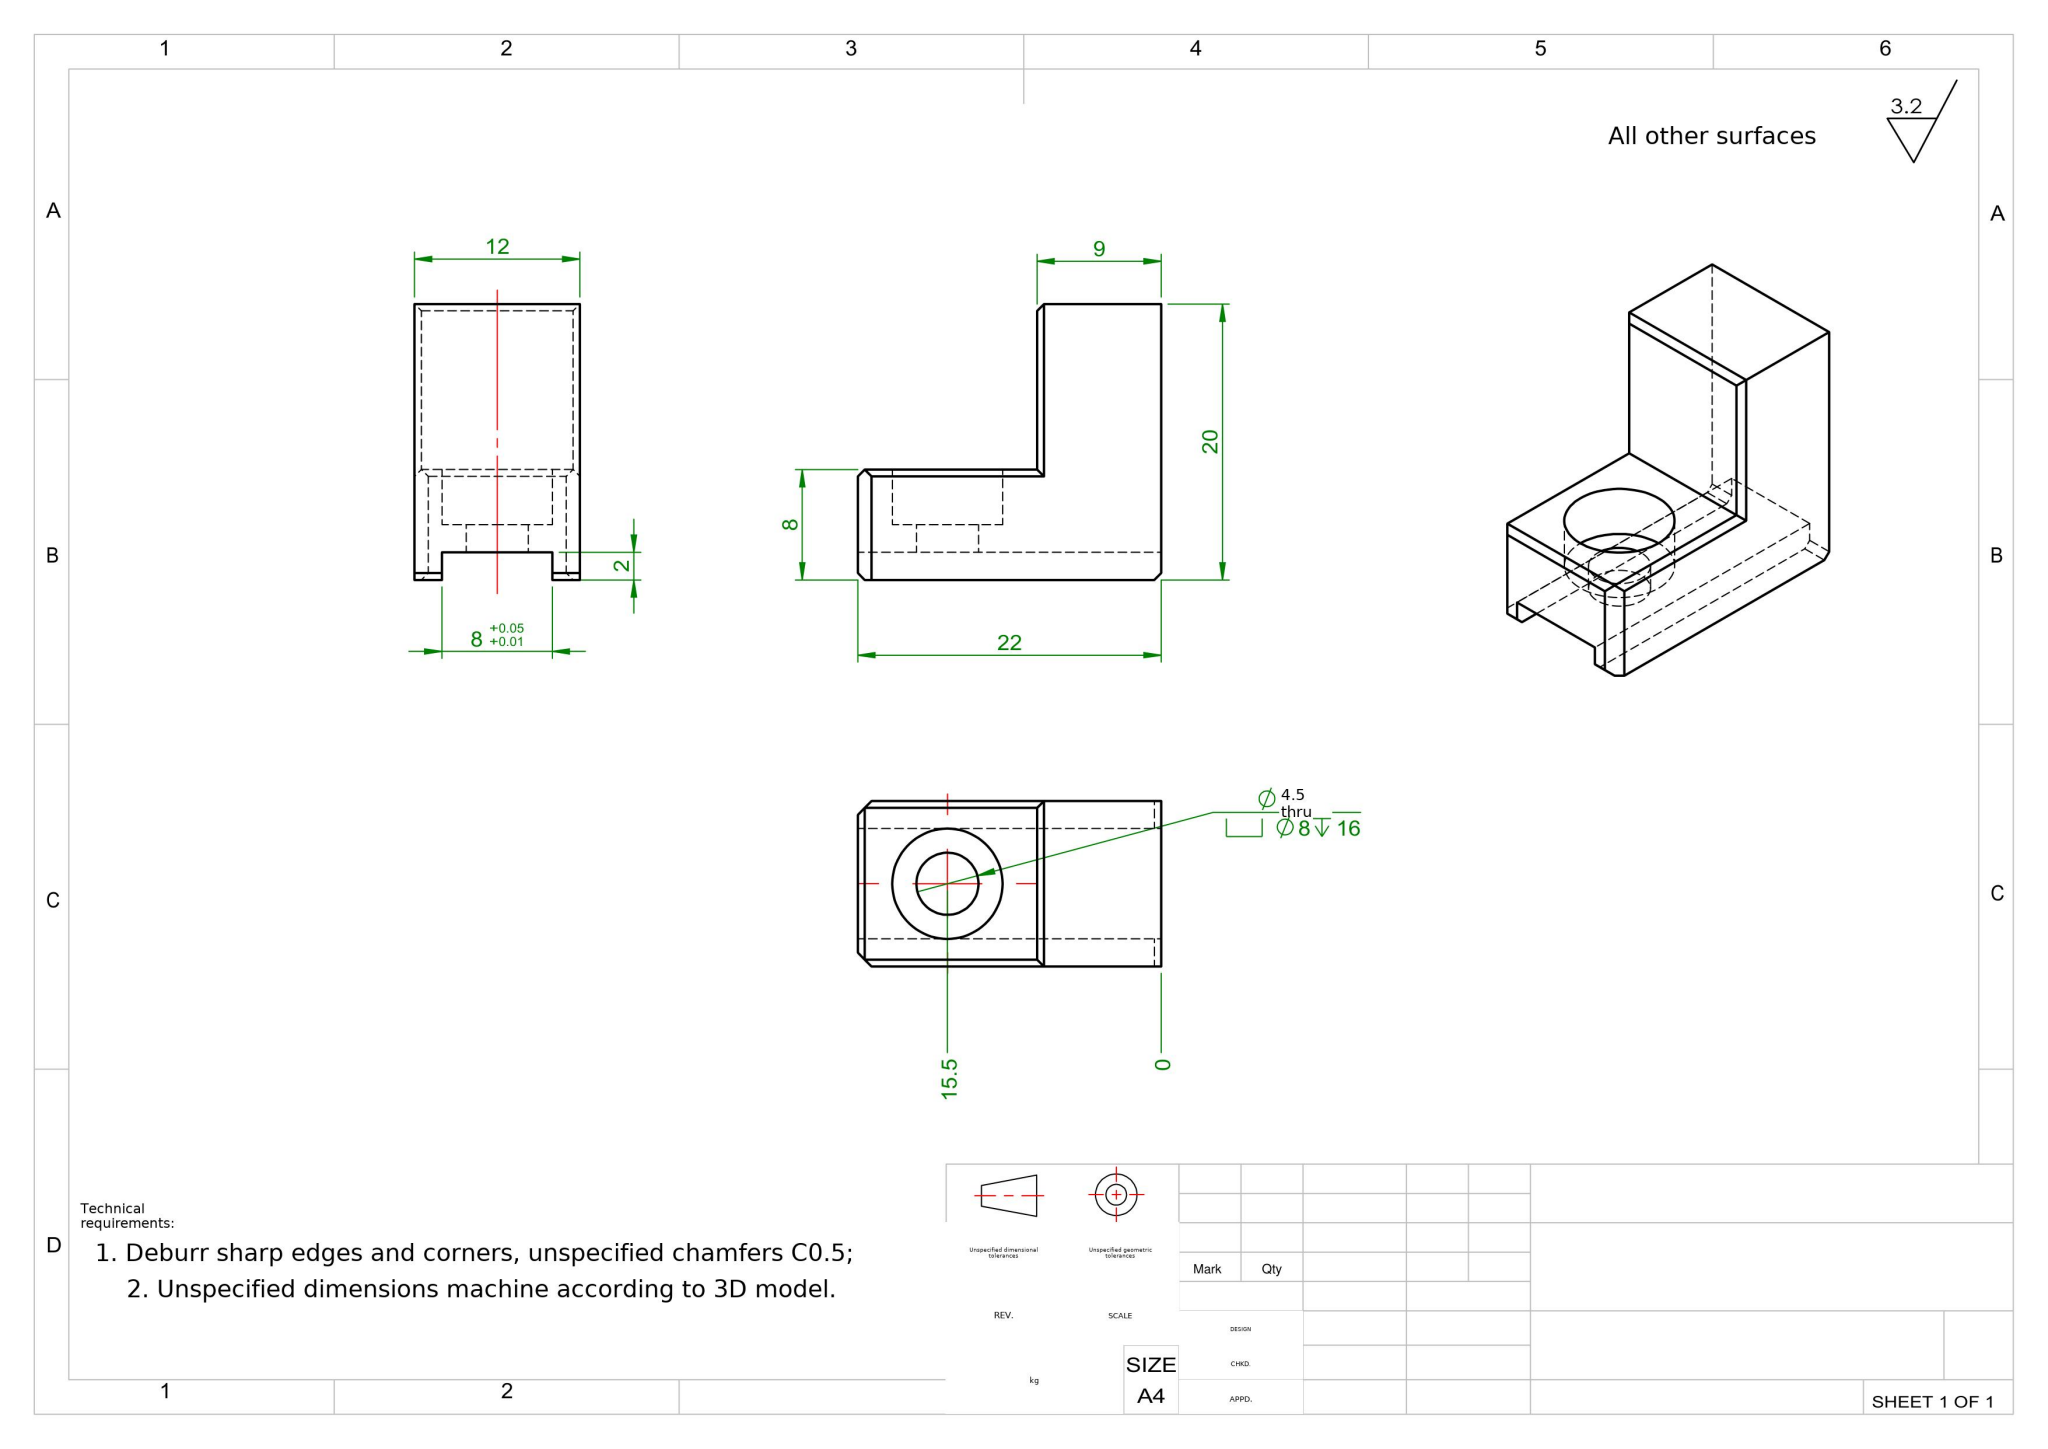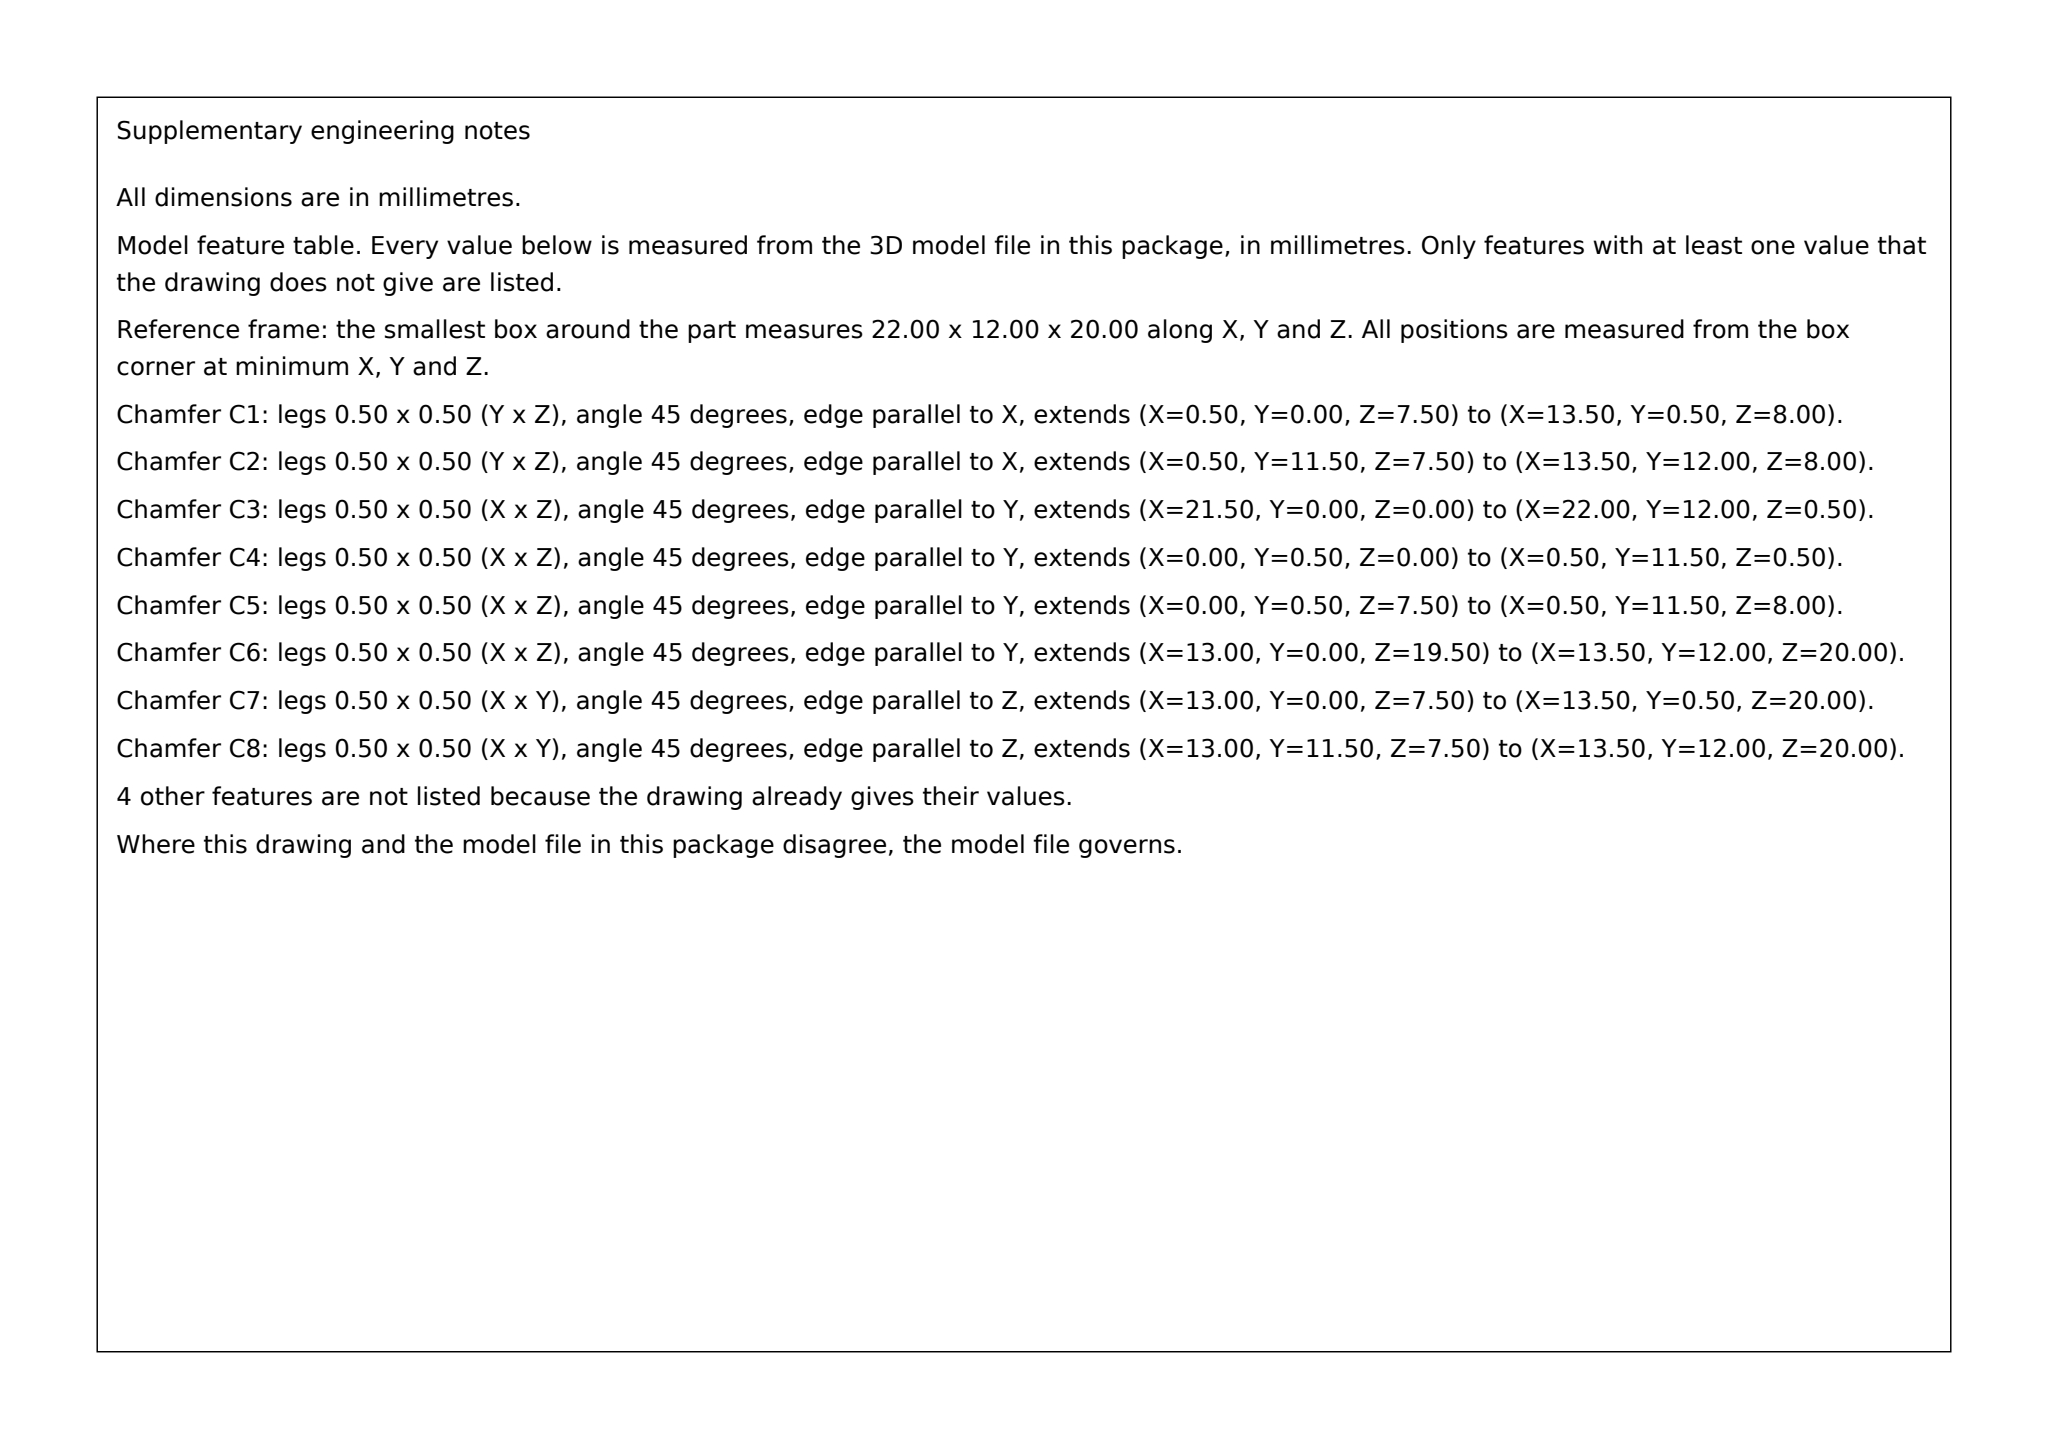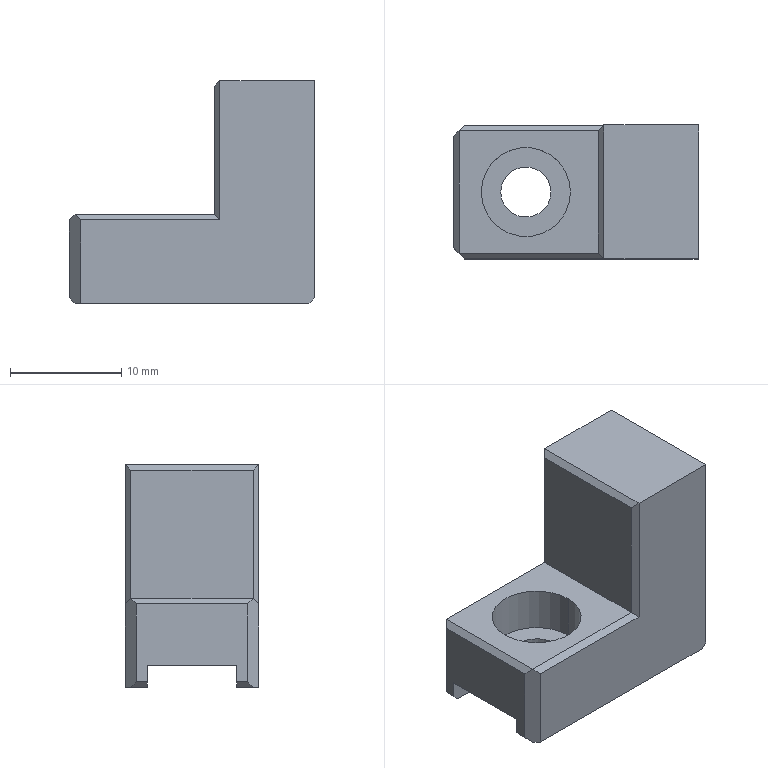Part | SolidWorks | mm | 1 solid | 29 faces | box 22 x 12 x 20 mm | volume 2806 mm3 | plane 25 | cylinder 4 | commonest cylinder face diameters 8 x2 4.5 x2
STEP:
#1=CARTESIAN_POINT('',(-8.5,0.,-6.));
#2=VERTEX_POINT('',#1);
#3=CARTESIAN_POINT('',(-0.5,0.,-6.));
#4=VERTEX_POINT('',#3);
#5=CARTESIAN_POINT('',(-4.5,0.,-6.));
#6=DIRECTION('',(0.,0.,1.));
#7=DIRECTION('',(1.,0.,0.));
#8=AXIS2_PLACEMENT_3D('',#5,#6,#7);
#9=CIRCLE('',#8,4.);
#10=EDGE_CURVE('',#2,#4,#9,.T.);
#11=ORIENTED_EDGE('',*,*,#10,.F.);
#12=CARTESIAN_POINT('',(-8.5,0.,-2.));
#13=VERTEX_POINT('',#12);
#14=CARTESIAN_POINT('',(-8.5,0.,10.));
#15=DIRECTION('',(0.,0.,1.));
#16=VECTOR('',#15,1000.);
#17=LINE('',#14,#16);
#18=EDGE_CURVE('',#2,#13,#17,.T.);
#19=ORIENTED_EDGE('',*,*,#18,.T.);
#20=CARTESIAN_POINT('',(-0.5,0.,-2.));
#21=VERTEX_POINT('',#20);
#22=CARTESIAN_POINT('',(-4.5,0.,-2.));
#23=DIRECTION('',(0.,0.,-1.));
#24=DIRECTION('',(-1.,0.,0.));
#25=AXIS2_PLACEMENT_3D('',#22,#23,#24);
#26=CIRCLE('',#25,4.);
#27=EDGE_CURVE('',#21,#13,#26,.T.);
#28=ORIENTED_EDGE('',*,*,#27,.F.);
#29=CARTESIAN_POINT('',(-0.5,0.,10.));
#30=DIRECTION('',(0.,0.,1.));
#31=VECTOR('',#30,1000.);
#32=LINE('',#29,#31);
#33=EDGE_CURVE('',#4,#21,#32,.T.);
#34=ORIENTED_EDGE('',*,*,#33,.F.);
#35=EDGE_LOOP('',(#11,#19,#28,#34));
#36=FACE_OUTER_BOUND('',#35,.T.);
#37=CARTESIAN_POINT('',(-4.5,0.,10.));
#38=DIRECTION('',(0.,0.,1.));
#39=DIRECTION('',(1.,0.,0.));
#40=AXIS2_PLACEMENT_3D('',#37,#38,#39);
#41=CYLINDRICAL_SURFACE('',#40,4.);
#42=ADVANCED_FACE('',(#36),#41,.F.);
#43=CARTESIAN_POINT('',(-6.75,0.,-8.));
#44=VERTEX_POINT('',#43);
#45=CARTESIAN_POINT('',(-2.25,0.,-8.));
#46=VERTEX_POINT('',#45);
#47=CARTESIAN_POINT('',(-4.5,0.,-8.));
#48=DIRECTION('',(0.,0.,1.));
#49=DIRECTION('',(0.,-1.,0.));
#50=AXIS2_PLACEMENT_3D('',#47,#48,#49);
#51=CIRCLE('',#50,2.25);
#52=EDGE_CURVE('',#44,#46,#51,.T.);
#53=ORIENTED_EDGE('',*,*,#52,.F.);
#54=CARTESIAN_POINT('',(-6.75,0.,-6.));
#55=VERTEX_POINT('',#54);
#56=CARTESIAN_POINT('',(-6.75,0.,10.));
#57=DIRECTION('',(0.,0.,1.));
#58=VECTOR('',#57,1000.);
#59=LINE('',#56,#58);
#60=EDGE_CURVE('',#44,#55,#59,.T.);
#61=ORIENTED_EDGE('',*,*,#60,.T.);
#62=CARTESIAN_POINT('',(-2.25,0.,-6.));
#63=VERTEX_POINT('',#62);
#64=CARTESIAN_POINT('',(-4.5,0.,-6.));
#65=DIRECTION('',(0.,0.,1.));
#66=DIRECTION('',(1.,0.,0.));
#67=AXIS2_PLACEMENT_3D('',#64,#65,#66);
#68=CIRCLE('',#67,2.25);
#69=EDGE_CURVE('',#55,#63,#68,.T.);
#70=ORIENTED_EDGE('',*,*,#69,.T.);
#71=CARTESIAN_POINT('',(-2.25,0.,10.));
#72=DIRECTION('',(0.,0.,1.));
#73=VECTOR('',#72,1000.);
#74=LINE('',#71,#73);
#75=EDGE_CURVE('',#46,#63,#74,.T.);
#76=ORIENTED_EDGE('',*,*,#75,.F.);
#77=EDGE_LOOP('',(#53,#61,#70,#76));
#78=FACE_OUTER_BOUND('',#77,.T.);
#79=CARTESIAN_POINT('',(-4.5,0.,10.));
#80=DIRECTION('',(0.,0.,1.));
#81=DIRECTION('',(1.,0.,0.));
#82=AXIS2_PLACEMENT_3D('',#79,#80,#81);
#83=CYLINDRICAL_SURFACE('',#82,2.25);
#84=ADVANCED_FACE('',(#78),#83,.F.);
#85=CARTESIAN_POINT('',(-10.,-6.,-10.));
#86=VERTEX_POINT('',#85);
#87=CARTESIAN_POINT('',(10.5,-6.,-10.));
#88=VERTEX_POINT('',#87);
#89=CARTESIAN_POINT('',(-11.,-6.,-10.));
#90=DIRECTION('',(1.,0.,0.));
#91=VECTOR('',#90,1000.);
#92=LINE('',#89,#91);
#93=EDGE_CURVE('',#86,#88,#92,.T.);
#94=ORIENTED_EDGE('',*,*,#93,.F.);
#95=CARTESIAN_POINT('',(-10.5,-5.5,-10.));
#96=VERTEX_POINT('',#95);
#97=CARTESIAN_POINT('',(-8.,-8.,-10.));
#98=DIRECTION('',(-0.7071,0.7071,0.));
#99=VECTOR('',#98,1000.);
#100=LINE('',#97,#99);
#101=EDGE_CURVE('',#86,#96,#100,.T.);
#102=ORIENTED_EDGE('',*,*,#101,.T.);
#103=CARTESIAN_POINT('',(-10.5,-4.,-10.));
#104=VERTEX_POINT('',#103);
#105=CARTESIAN_POINT('',(-10.5,-4.,-10.));
#106=DIRECTION('',(0.,1.,0.));
#107=VECTOR('',#106,1000.);
#108=LINE('',#105,#107);
#109=EDGE_CURVE('',#96,#104,#108,.T.);
#110=ORIENTED_EDGE('',*,*,#109,.T.);
#111=CARTESIAN_POINT('',(10.5,-4.,-10.));
#112=VERTEX_POINT('',#111);
#113=CARTESIAN_POINT('',(0.,-4.,-10.));
#114=DIRECTION('',(-1.,0.,0.));
#115=VECTOR('',#114,1000.);
#116=LINE('',#113,#115);
#117=EDGE_CURVE('',#112,#104,#116,.T.);
#118=ORIENTED_EDGE('',*,*,#117,.F.);
#119=CARTESIAN_POINT('',(10.5,-6.,-10.));
#120=DIRECTION('',(0.,-1.,0.));
#121=VECTOR('',#120,1000.);
#122=LINE('',#119,#121);
#123=EDGE_CURVE('',#112,#88,#122,.T.);
#124=ORIENTED_EDGE('',*,*,#123,.T.);
#125=EDGE_LOOP('',(#94,#102,#110,#118,#124));
#126=FACE_OUTER_BOUND('',#125,.T.);
#127=CARTESIAN_POINT('',(0.,0.,-10.));
#128=DIRECTION('',(0.,0.,-1.));
#129=DIRECTION('',(-1.,0.,0.));
#130=AXIS2_PLACEMENT_3D('',#127,#128,#129);
#131=PLANE('',#130);
#132=ADVANCED_FACE('',(#126),#131,.T.);
#133=CARTESIAN_POINT('',(11.,4.,-8.));
#134=VERTEX_POINT('',#133);
#135=CARTESIAN_POINT('',(11.,4.,-9.5));
#136=VERTEX_POINT('',#135);
#137=CARTESIAN_POINT('',(11.,4.,-12.));
#138=DIRECTION('',(0.,0.,-1.));
#139=VECTOR('',#138,1000.);
#140=LINE('',#137,#139);
#141=EDGE_CURVE('',#134,#136,#140,.T.);
#142=ORIENTED_EDGE('',*,*,#141,.T.);
#143=CARTESIAN_POINT('',(11.,6.,-9.5));
#144=VERTEX_POINT('',#143);
#145=CARTESIAN_POINT('',(11.,6.,-9.5));
#146=DIRECTION('',(0.,1.,0.));
#147=VECTOR('',#146,1000.);
#148=LINE('',#145,#147);
#149=EDGE_CURVE('',#136,#144,#148,.T.);
#150=ORIENTED_EDGE('',*,*,#149,.T.);
#151=CARTESIAN_POINT('',(11.,6.,10.));
#152=VERTEX_POINT('',#151);
#153=CARTESIAN_POINT('',(11.,6.,10.));
#154=DIRECTION('',(0.,0.,-1.));
#155=VECTOR('',#154,1000.);
#156=LINE('',#153,#155);
#157=EDGE_CURVE('',#152,#144,#156,.T.);
#158=ORIENTED_EDGE('',*,*,#157,.F.);
#159=CARTESIAN_POINT('',(11.,-6.,10.));
#160=VERTEX_POINT('',#159);
#161=CARTESIAN_POINT('',(11.,-6.,10.));
#162=DIRECTION('',(0.,1.,0.));
#163=VECTOR('',#162,1000.);
#164=LINE('',#161,#163);
#165=EDGE_CURVE('',#160,#152,#164,.T.);
#166=ORIENTED_EDGE('',*,*,#165,.F.);
#167=CARTESIAN_POINT('',(11.,-6.,-9.5));
#168=VERTEX_POINT('',#167);
#169=CARTESIAN_POINT('',(11.,-6.,10.));
#170=DIRECTION('',(0.,0.,-1.));
#171=VECTOR('',#170,1000.);
#172=LINE('',#169,#171);
#173=EDGE_CURVE('',#160,#168,#172,.T.);
#174=ORIENTED_EDGE('',*,*,#173,.T.);
#175=CARTESIAN_POINT('',(11.,-4.,-9.5));
#176=VERTEX_POINT('',#175);
#177=CARTESIAN_POINT('',(11.,-4.,-9.5));
#178=DIRECTION('',(0.,1.,0.));
#179=VECTOR('',#178,1000.);
#180=LINE('',#177,#179);
#181=EDGE_CURVE('',#168,#176,#180,.T.);
#182=ORIENTED_EDGE('',*,*,#181,.T.);
#183=CARTESIAN_POINT('',(11.,-4.,-8.));
#184=VERTEX_POINT('',#183);
#185=CARTESIAN_POINT('',(11.,-4.,-12.));
#186=DIRECTION('',(0.,0.,1.));
#187=VECTOR('',#186,1000.);
#188=LINE('',#185,#187);
#189=EDGE_CURVE('',#176,#184,#188,.T.);
#190=ORIENTED_EDGE('',*,*,#189,.T.);
#191=CARTESIAN_POINT('',(11.,4.,-8.));
#192=DIRECTION('',(0.,1.,-0.));
#193=VECTOR('',#192,1000.);
#194=LINE('',#191,#193);
#195=EDGE_CURVE('',#184,#134,#194,.T.);
#196=ORIENTED_EDGE('',*,*,#195,.T.);
#197=EDGE_LOOP('',(#142,#150,#158,#166,#174,#182,#190,#196));
#198=FACE_OUTER_BOUND('',#197,.T.);
#199=CARTESIAN_POINT('',(11.,-6.,10.));
#200=DIRECTION('',(-1.,0.,0.));
#201=DIRECTION('',(0.,0.,1.));
#202=AXIS2_PLACEMENT_3D('',#199,#200,#201);
#203=PLANE('',#202);
#204=ADVANCED_FACE('',(#198),#203,.F.);
#205=CARTESIAN_POINT('',(10.5,6.,-10.));
#206=VERTEX_POINT('',#205);
#207=CARTESIAN_POINT('',(-10.,6.,-10.));
#208=VERTEX_POINT('',#207);
#209=CARTESIAN_POINT('',(-11.,6.,-10.));
#210=DIRECTION('',(-1.,0.,0.));
#211=VECTOR('',#210,1000.);
#212=LINE('',#209,#211);
#213=EDGE_CURVE('',#206,#208,#212,.T.);
#214=ORIENTED_EDGE('',*,*,#213,.T.);
#215=CARTESIAN_POINT('',(-10.,6.,-2.5));
#216=VERTEX_POINT('',#215);
#217=CARTESIAN_POINT('',(-10.,6.,10.));
#218=DIRECTION('',(0.,0.,1.));
#219=VECTOR('',#218,1000.);
#220=LINE('',#217,#219);
#221=EDGE_CURVE('',#208,#216,#220,.T.);
#222=ORIENTED_EDGE('',*,*,#221,.T.);
#223=CARTESIAN_POINT('',(2.5,6.,-2.5));
#224=VERTEX_POINT('',#223);
#225=CARTESIAN_POINT('',(-11.,6.,-2.5));
#226=DIRECTION('',(1.,0.,0.));
#227=VECTOR('',#226,1000.);
#228=LINE('',#225,#227);
#229=EDGE_CURVE('',#216,#224,#228,.T.);
#230=ORIENTED_EDGE('',*,*,#229,.T.);
#231=CARTESIAN_POINT('',(2.5,6.,10.));
#232=VERTEX_POINT('',#231);
#233=CARTESIAN_POINT('',(2.5,6.,10.));
#234=DIRECTION('',(-0.,0.,1.));
#235=VECTOR('',#234,1000.);
#236=LINE('',#233,#235);
#237=EDGE_CURVE('',#224,#232,#236,.T.);
#238=ORIENTED_EDGE('',*,*,#237,.T.);
#239=CARTESIAN_POINT('',(-11.,6.,10.));
#240=DIRECTION('',(-1.,0.,0.));
#241=VECTOR('',#240,1000.);
#242=LINE('',#239,#241);
#243=EDGE_CURVE('',#152,#232,#242,.T.);
#244=ORIENTED_EDGE('',*,*,#243,.F.);
#245=ORIENTED_EDGE('',*,*,#157,.T.);
#246=CARTESIAN_POINT('',(11.,6.,-9.5));
#247=DIRECTION('',(-0.7071,0.,-0.7071));
#248=VECTOR('',#247,1000.);
#249=LINE('',#246,#248);
#250=EDGE_CURVE('',#144,#206,#249,.T.);
#251=ORIENTED_EDGE('',*,*,#250,.T.);
#252=EDGE_LOOP('',(#214,#222,#230,#238,#244,#245,#251));
#253=FACE_OUTER_BOUND('',#252,.T.);
#254=CARTESIAN_POINT('',(-11.,6.,10.));
#255=DIRECTION('',(0.,-1.,0.));
#256=DIRECTION('',(0.,0.,-1.));
#257=AXIS2_PLACEMENT_3D('',#254,#255,#256);
#258=PLANE('',#257);
#259=ADVANCED_FACE('',(#253),#258,.F.);
#260=CARTESIAN_POINT('',(-11.,-5.,-2.5));
#261=VERTEX_POINT('',#260);
#262=CARTESIAN_POINT('',(-11.,5.,-2.5));
#263=VERTEX_POINT('',#262);
#264=CARTESIAN_POINT('',(-11.,-6.,-2.5));
#265=DIRECTION('',(0.,1.,0.));
#266=VECTOR('',#265,1000.);
#267=LINE('',#264,#266);
#268=EDGE_CURVE('',#261,#263,#267,.T.);
#269=ORIENTED_EDGE('',*,*,#268,.T.);
#270=CARTESIAN_POINT('',(-11.,5.,-9.5));
#271=VERTEX_POINT('',#270);
#272=CARTESIAN_POINT('',(-11.,5.,10.));
#273=DIRECTION('',(0.,0.,-1.));
#274=VECTOR('',#273,1000.);
#275=LINE('',#272,#274);
#276=EDGE_CURVE('',#263,#271,#275,.T.);
#277=ORIENTED_EDGE('',*,*,#276,.T.);
#278=CARTESIAN_POINT('',(-11.,4.,-9.5));
#279=VERTEX_POINT('',#278);
#280=CARTESIAN_POINT('',(-11.,4.,-9.5));
#281=DIRECTION('',(0.,-1.,0.));
#282=VECTOR('',#281,1000.);
#283=LINE('',#280,#282);
#284=EDGE_CURVE('',#271,#279,#283,.T.);
#285=ORIENTED_EDGE('',*,*,#284,.T.);
#286=CARTESIAN_POINT('',(-11.,4.,-8.));
#287=VERTEX_POINT('',#286);
#288=CARTESIAN_POINT('',(-11.,4.,-12.));
#289=DIRECTION('',(0.,0.,-1.));
#290=VECTOR('',#289,1000.);
#291=LINE('',#288,#290);
#292=EDGE_CURVE('',#287,#279,#291,.T.);
#293=ORIENTED_EDGE('',*,*,#292,.F.);
#294=CARTESIAN_POINT('',(-11.,-4.,-8.));
#295=VERTEX_POINT('',#294);
#296=CARTESIAN_POINT('',(-11.,4.,-8.));
#297=DIRECTION('',(0.,1.,-0.));
#298=VECTOR('',#297,1000.);
#299=LINE('',#296,#298);
#300=EDGE_CURVE('',#295,#287,#299,.T.);
#301=ORIENTED_EDGE('',*,*,#300,.F.);
#302=CARTESIAN_POINT('',(-11.,-4.,-9.5));
#303=VERTEX_POINT('',#302);
#304=CARTESIAN_POINT('',(-11.,-4.,-12.));
#305=DIRECTION('',(0.,0.,1.));
#306=VECTOR('',#305,1000.);
#307=LINE('',#304,#306);
#308=EDGE_CURVE('',#303,#295,#307,.T.);
#309=ORIENTED_EDGE('',*,*,#308,.F.);
#310=CARTESIAN_POINT('',(-11.,-5.,-9.5));
#311=VERTEX_POINT('',#310);
#312=CARTESIAN_POINT('',(-11.,-6.,-9.5));
#313=DIRECTION('',(0.,-1.,0.));
#314=VECTOR('',#313,1000.);
#315=LINE('',#312,#314);
#316=EDGE_CURVE('',#303,#311,#315,.T.);
#317=ORIENTED_EDGE('',*,*,#316,.T.);
#318=CARTESIAN_POINT('',(-11.,-5.,10.));
#319=DIRECTION('',(0.,0.,1.));
#320=VECTOR('',#319,1000.);
#321=LINE('',#318,#320);
#322=EDGE_CURVE('',#311,#261,#321,.T.);
#323=ORIENTED_EDGE('',*,*,#322,.T.);
#324=EDGE_LOOP('',(#269,#277,#285,#293,#301,#309,#317,#323));
#325=FACE_OUTER_BOUND('',#324,.T.);
#326=CARTESIAN_POINT('',(-11.,-6.,10.));
#327=DIRECTION('',(1.,0.,0.));
#328=DIRECTION('',(0.,0.,-1.));
#329=AXIS2_PLACEMENT_3D('',#326,#327,#328);
#330=PLANE('',#329);
#331=ADVANCED_FACE('',(#325),#330,.F.);
#332=CARTESIAN_POINT('',(2.5,-6.,-2.5));
#333=VERTEX_POINT('',#332);
#334=CARTESIAN_POINT('',(-10.,-6.,-2.5));
#335=VERTEX_POINT('',#334);
#336=CARTESIAN_POINT('',(-11.,-6.,-2.5));
#337=DIRECTION('',(-1.,0.,0.));
#338=VECTOR('',#337,1000.);
#339=LINE('',#336,#338);
#340=EDGE_CURVE('',#333,#335,#339,.T.);
#341=ORIENTED_EDGE('',*,*,#340,.T.);
#342=CARTESIAN_POINT('',(-10.,-6.,10.));
#343=DIRECTION('',(0.,0.,-1.));
#344=VECTOR('',#343,1000.);
#345=LINE('',#342,#344);
#346=EDGE_CURVE('',#335,#86,#345,.T.);
#347=ORIENTED_EDGE('',*,*,#346,.T.);
#348=ORIENTED_EDGE('',*,*,#93,.T.);
#349=CARTESIAN_POINT('',(11.,-6.,-9.5));
#350=DIRECTION('',(0.7071,0.,0.7071));
#351=VECTOR('',#350,1000.);
#352=LINE('',#349,#351);
#353=EDGE_CURVE('',#88,#168,#352,.T.);
#354=ORIENTED_EDGE('',*,*,#353,.T.);
#355=ORIENTED_EDGE('',*,*,#173,.F.);
#356=CARTESIAN_POINT('',(2.5,-6.,10.));
#357=VERTEX_POINT('',#356);
#358=CARTESIAN_POINT('',(-11.,-6.,10.));
#359=DIRECTION('',(1.,0.,0.));
#360=VECTOR('',#359,1000.);
#361=LINE('',#358,#360);
#362=EDGE_CURVE('',#357,#160,#361,.T.);
#363=ORIENTED_EDGE('',*,*,#362,.F.);
#364=CARTESIAN_POINT('',(2.5,-6.,10.));
#365=DIRECTION('',(0.,0.,-1.));
#366=VECTOR('',#365,1000.);
#367=LINE('',#364,#366);
#368=EDGE_CURVE('',#357,#333,#367,.T.);
#369=ORIENTED_EDGE('',*,*,#368,.T.);
#370=EDGE_LOOP('',(#341,#347,#348,#354,#355,#363,#369));
#371=FACE_OUTER_BOUND('',#370,.T.);
#372=CARTESIAN_POINT('',(-11.,-6.,10.));
#373=DIRECTION('',(0.,1.,0.));
#374=DIRECTION('',(0.,0.,1.));
#375=AXIS2_PLACEMENT_3D('',#372,#373,#374);
#376=PLANE('',#375);
#377=ADVANCED_FACE('',(#371),#376,.F.);
#378=ORIENTED_EDGE('',*,*,#243,.T.);
#379=CARTESIAN_POINT('',(2.5,0.,10.));
#380=DIRECTION('',(0.,-1.,0.));
#381=VECTOR('',#380,1000.);
#382=LINE('',#379,#381);
#383=EDGE_CURVE('',#232,#357,#382,.T.);
#384=ORIENTED_EDGE('',*,*,#383,.T.);
#385=ORIENTED_EDGE('',*,*,#362,.T.);
#386=ORIENTED_EDGE('',*,*,#165,.T.);
#387=EDGE_LOOP('',(#378,#384,#385,#386));
#388=FACE_OUTER_BOUND('',#387,.T.);
#389=CARTESIAN_POINT('',(0.,0.,10.));
#390=DIRECTION('',(0.,0.,-1.));
#391=DIRECTION('',(-1.,0.,0.));
#392=AXIS2_PLACEMENT_3D('',#389,#390,#391);
#393=PLANE('',#392);
#394=ADVANCED_FACE('',(#388),#393,.F.);
#395=CARTESIAN_POINT('',(-10.5,4.,-10.));
#396=VERTEX_POINT('',#395);
#397=CARTESIAN_POINT('',(-10.5,5.5,-10.));
#398=VERTEX_POINT('',#397);
#399=CARTESIAN_POINT('',(-10.5,6.,-10.));
#400=DIRECTION('',(0.,1.,0.));
#401=VECTOR('',#400,1000.);
#402=LINE('',#399,#401);
#403=EDGE_CURVE('',#396,#398,#402,.T.);
#404=ORIENTED_EDGE('',*,*,#403,.T.);
#405=CARTESIAN_POINT('',(-8.,8.,-10.));
#406=DIRECTION('',(0.7071,0.7071,0.));
#407=VECTOR('',#406,1000.);
#408=LINE('',#405,#407);
#409=EDGE_CURVE('',#398,#208,#408,.T.);
#410=ORIENTED_EDGE('',*,*,#409,.T.);
#411=ORIENTED_EDGE('',*,*,#213,.F.);
#412=CARTESIAN_POINT('',(10.5,4.,-10.));
#413=VERTEX_POINT('',#412);
#414=CARTESIAN_POINT('',(10.5,4.,-10.));
#415=DIRECTION('',(0.,-1.,0.));
#416=VECTOR('',#415,1000.);
#417=LINE('',#414,#416);
#418=EDGE_CURVE('',#206,#413,#417,.T.);
#419=ORIENTED_EDGE('',*,*,#418,.T.);
#420=CARTESIAN_POINT('',(0.,4.,-10.));
#421=DIRECTION('',(1.,0.,0.));
#422=VECTOR('',#421,1000.);
#423=LINE('',#420,#422);
#424=EDGE_CURVE('',#396,#413,#423,.T.);
#425=ORIENTED_EDGE('',*,*,#424,.F.);
#426=EDGE_LOOP('',(#404,#410,#411,#419,#425));
#427=FACE_OUTER_BOUND('',#426,.T.);
#428=CARTESIAN_POINT('',(0.,0.,-10.));
#429=DIRECTION('',(0.,0.,-1.));
#430=DIRECTION('',(-1.,0.,0.));
#431=AXIS2_PLACEMENT_3D('',#428,#429,#430);
#432=PLANE('',#431);
#433=ADVANCED_FACE('',(#427),#432,.T.);
#434=CARTESIAN_POINT('',(-4.5,0.,-8.));
#435=DIRECTION('',(0.,0.,1.));
#436=DIRECTION('',(0.,-1.,0.));
#437=AXIS2_PLACEMENT_3D('',#434,#435,#436);
#438=CIRCLE('',#437,2.25);
#439=EDGE_CURVE('',#46,#44,#438,.T.);
#440=ORIENTED_EDGE('',*,*,#439,.T.);
#441=ORIENTED_EDGE('',*,*,#52,.T.);
#442=EDGE_LOOP('',(#440,#441));
#443=FACE_BOUND('',#442,.T.);
#444=ORIENTED_EDGE('',*,*,#300,.T.);
#445=CARTESIAN_POINT('',(11.,4.,-8.));
#446=DIRECTION('',(-1.,0.,0.));
#447=VECTOR('',#446,1000.);
#448=LINE('',#445,#447);
#449=EDGE_CURVE('',#134,#287,#448,.T.);
#450=ORIENTED_EDGE('',*,*,#449,.F.);
#451=ORIENTED_EDGE('',*,*,#195,.F.);
#452=CARTESIAN_POINT('',(11.,-4.,-8.));
#453=DIRECTION('',(-1.,0.,0.));
#454=VECTOR('',#453,1000.);
#455=LINE('',#452,#454);
#456=EDGE_CURVE('',#184,#295,#455,.T.);
#457=ORIENTED_EDGE('',*,*,#456,.T.);
#458=EDGE_LOOP('',(#444,#450,#451,#457));
#459=FACE_OUTER_BOUND('',#458,.T.);
#460=CARTESIAN_POINT('',(11.,4.,-8.));
#461=DIRECTION('',(0.,0.,1.));
#462=DIRECTION('',(0.,-1.,0.));
#463=AXIS2_PLACEMENT_3D('',#460,#461,#462);
#464=PLANE('',#463);
#465=ADVANCED_FACE('',(#443,#459),#464,.F.);
#466=ORIENTED_EDGE('',*,*,#189,.F.);
#467=CARTESIAN_POINT('',(11.,-4.,-9.5));
#468=DIRECTION('',(-0.7071,0.,-0.7071));
#469=VECTOR('',#468,1000.);
#470=LINE('',#467,#469);
#471=EDGE_CURVE('',#176,#112,#470,.T.);
#472=ORIENTED_EDGE('',*,*,#471,.T.);
#473=ORIENTED_EDGE('',*,*,#117,.T.);
#474=CARTESIAN_POINT('',(-11.,-4.,-9.5));
#475=DIRECTION('',(-0.7071,0.,0.7071));
#476=VECTOR('',#475,1000.);
#477=LINE('',#474,#476);
#478=EDGE_CURVE('',#104,#303,#477,.T.);
#479=ORIENTED_EDGE('',*,*,#478,.T.);
#480=ORIENTED_EDGE('',*,*,#308,.T.);
#481=ORIENTED_EDGE('',*,*,#456,.F.);
#482=EDGE_LOOP('',(#466,#472,#473,#479,#480,#481));
#483=FACE_OUTER_BOUND('',#482,.T.);
#484=CARTESIAN_POINT('',(11.,-4.,-12.));
#485=DIRECTION('',(0.,-1.,0.));
#486=DIRECTION('',(0.,0.,-1.));
#487=AXIS2_PLACEMENT_3D('',#484,#485,#486);
#488=PLANE('',#487);
#489=ADVANCED_FACE('',(#483),#488,.F.);
#490=ORIENTED_EDGE('',*,*,#424,.T.);
#491=CARTESIAN_POINT('',(11.,4.,-9.5));
#492=DIRECTION('',(0.7071,0.,0.7071));
#493=VECTOR('',#492,1000.);
#494=LINE('',#491,#493);
#495=EDGE_CURVE('',#413,#136,#494,.T.);
#496=ORIENTED_EDGE('',*,*,#495,.T.);
#497=ORIENTED_EDGE('',*,*,#141,.F.);
#498=ORIENTED_EDGE('',*,*,#449,.T.);
#499=ORIENTED_EDGE('',*,*,#292,.T.);
#500=CARTESIAN_POINT('',(-11.,4.,-9.5));
#501=DIRECTION('',(0.7071,0.,-0.7071));
#502=VECTOR('',#501,1000.);
#503=LINE('',#500,#502);
#504=EDGE_CURVE('',#279,#396,#503,.T.);
#505=ORIENTED_EDGE('',*,*,#504,.T.);
#506=EDGE_LOOP('',(#490,#496,#497,#498,#499,#505));
#507=FACE_OUTER_BOUND('',#506,.T.);
#508=CARTESIAN_POINT('',(11.,4.,-12.));
#509=DIRECTION('',(0.,1.,0.));
#510=DIRECTION('',(0.,0.,1.));
#511=AXIS2_PLACEMENT_3D('',#508,#509,#510);
#512=PLANE('',#511);
#513=ADVANCED_FACE('',(#507),#512,.F.);
#514=CARTESIAN_POINT('',(2.,-5.5,9.5));
#515=VERTEX_POINT('',#514);
#516=CARTESIAN_POINT('',(2.,5.5,9.5));
#517=VERTEX_POINT('',#516);
#518=CARTESIAN_POINT('',(2.,6.,9.5));
#519=DIRECTION('',(0.,1.,0.));
#520=VECTOR('',#519,1000.);
#521=LINE('',#518,#520);
#522=EDGE_CURVE('',#515,#517,#521,.T.);
#523=ORIENTED_EDGE('',*,*,#522,.T.);
#524=CARTESIAN_POINT('',(2.,5.5,-2.));
#525=VERTEX_POINT('',#524);
#526=CARTESIAN_POINT('',(2.,5.5,10.));
#527=DIRECTION('',(0.,0.,-1.));
#528=VECTOR('',#527,1000.);
#529=LINE('',#526,#528);
#530=EDGE_CURVE('',#517,#525,#529,.T.);
#531=ORIENTED_EDGE('',*,*,#530,.T.);
#532=CARTESIAN_POINT('',(2.,-5.5,-2.));
#533=VERTEX_POINT('',#532);
#534=CARTESIAN_POINT('',(2.,6.,-2.));
#535=DIRECTION('',(0.,-1.,0.));
#536=VECTOR('',#535,1000.);
#537=LINE('',#534,#536);
#538=EDGE_CURVE('',#525,#533,#537,.T.);
#539=ORIENTED_EDGE('',*,*,#538,.T.);
#540=CARTESIAN_POINT('',(2.,-5.5,10.));
#541=DIRECTION('',(-0.,0.,1.));
#542=VECTOR('',#541,1000.);
#543=LINE('',#540,#542);
#544=EDGE_CURVE('',#533,#515,#543,.T.);
#545=ORIENTED_EDGE('',*,*,#544,.T.);
#546=EDGE_LOOP('',(#523,#531,#539,#545));
#547=FACE_OUTER_BOUND('',#546,.T.);
#548=CARTESIAN_POINT('',(2.,6.,10.));
#549=DIRECTION('',(1.,0.,0.));
#550=DIRECTION('',(0.,0.,-1.));
#551=AXIS2_PLACEMENT_3D('',#548,#549,#550);
#552=PLANE('',#551);
#553=ADVANCED_FACE('',(#547),#552,.F.);
#554=ORIENTED_EDGE('',*,*,#27,.T.);
#555=CARTESIAN_POINT('',(-4.5,0.,-2.));
#556=DIRECTION('',(0.,0.,-1.));
#557=DIRECTION('',(-1.,0.,0.));
#558=AXIS2_PLACEMENT_3D('',#555,#556,#557);
#559=CIRCLE('',#558,4.);
#560=EDGE_CURVE('',#13,#21,#559,.T.);
#561=ORIENTED_EDGE('',*,*,#560,.T.);
#562=EDGE_LOOP('',(#554,#561));
#563=FACE_BOUND('',#562,.T.);
#564=ORIENTED_EDGE('',*,*,#538,.F.);
#565=CARTESIAN_POINT('',(-10.5,5.5,-2.));
#566=VERTEX_POINT('',#565);
#567=CARTESIAN_POINT('',(-11.,5.5,-2.));
#568=DIRECTION('',(-1.,0.,0.));
#569=VECTOR('',#568,1000.);
#570=LINE('',#567,#569);
#571=EDGE_CURVE('',#525,#566,#570,.T.);
#572=ORIENTED_EDGE('',*,*,#571,.T.);
#573=CARTESIAN_POINT('',(-10.5,-5.5,-2.));
#574=VERTEX_POINT('',#573);
#575=CARTESIAN_POINT('',(-10.5,6.,-2.));
#576=DIRECTION('',(0.,-1.,0.));
#577=VECTOR('',#576,1000.);
#578=LINE('',#575,#577);
#579=EDGE_CURVE('',#566,#574,#578,.T.);
#580=ORIENTED_EDGE('',*,*,#579,.T.);
#581=CARTESIAN_POINT('',(-11.,-5.5,-2.));
#582=DIRECTION('',(1.,0.,0.));
#583=VECTOR('',#582,1000.);
#584=LINE('',#581,#583);
#585=EDGE_CURVE('',#574,#533,#584,.T.);
#586=ORIENTED_EDGE('',*,*,#585,.T.);
#587=EDGE_LOOP('',(#564,#572,#580,#586));
#588=FACE_OUTER_BOUND('',#587,.T.);
#589=CARTESIAN_POINT('',(-11.,6.,-2.));
#590=DIRECTION('',(0.,0.,-1.));
#591=DIRECTION('',(-1.,0.,0.));
#592=AXIS2_PLACEMENT_3D('',#589,#590,#591);
#593=PLANE('',#592);
#594=ADVANCED_FACE('',(#563,#588),#593,.F.);
#595=ORIENTED_EDGE('',*,*,#60,.F.);
#596=ORIENTED_EDGE('',*,*,#439,.F.);
#597=ORIENTED_EDGE('',*,*,#75,.T.);
#598=CARTESIAN_POINT('',(-4.5,0.,-6.));
#599=DIRECTION('',(0.,0.,1.));
#600=DIRECTION('',(1.,0.,0.));
#601=AXIS2_PLACEMENT_3D('',#598,#599,#600);
#602=CIRCLE('',#601,2.25);
#603=EDGE_CURVE('',#63,#55,#602,.T.);
#604=ORIENTED_EDGE('',*,*,#603,.T.);
#605=EDGE_LOOP('',(#595,#596,#597,#604));
#606=FACE_OUTER_BOUND('',#605,.T.);
#607=CARTESIAN_POINT('',(-4.5,0.,10.));
#608=DIRECTION('',(0.,0.,1.));
#609=DIRECTION('',(1.,0.,0.));
#610=AXIS2_PLACEMENT_3D('',#607,#608,#609);
#611=CYLINDRICAL_SURFACE('',#610,2.25);
#612=ADVANCED_FACE('',(#606),#611,.F.);
#613=ORIENTED_EDGE('',*,*,#18,.F.);
#614=CARTESIAN_POINT('',(-4.5,0.,-6.));
#615=DIRECTION('',(0.,0.,1.));
#616=DIRECTION('',(1.,0.,0.));
#617=AXIS2_PLACEMENT_3D('',#614,#615,#616);
#618=CIRCLE('',#617,4.);
#619=EDGE_CURVE('',#4,#2,#618,.T.);
#620=ORIENTED_EDGE('',*,*,#619,.F.);
#621=ORIENTED_EDGE('',*,*,#33,.T.);
#622=ORIENTED_EDGE('',*,*,#560,.F.);
#623=EDGE_LOOP('',(#613,#620,#621,#622));
#624=FACE_OUTER_BOUND('',#623,.T.);
#625=CARTESIAN_POINT('',(-4.5,0.,10.));
#626=DIRECTION('',(0.,0.,1.));
#627=DIRECTION('',(1.,0.,0.));
#628=AXIS2_PLACEMENT_3D('',#625,#626,#627);
#629=CYLINDRICAL_SURFACE('',#628,4.);
#630=ADVANCED_FACE('',(#624),#629,.F.);
#631=ORIENTED_EDGE('',*,*,#603,.F.);
#632=ORIENTED_EDGE('',*,*,#69,.F.);
#633=EDGE_LOOP('',(#631,#632));
#634=FACE_BOUND('',#633,.T.);
#635=ORIENTED_EDGE('',*,*,#619,.T.);
#636=ORIENTED_EDGE('',*,*,#10,.T.);
#637=EDGE_LOOP('',(#635,#636));
#638=FACE_OUTER_BOUND('',#637,.T.);
#639=CARTESIAN_POINT('',(-2.25,0.,-6.));
#640=DIRECTION('',(0.,0.,-1.));
#641=DIRECTION('',(-1.,0.,0.));
#642=AXIS2_PLACEMENT_3D('',#639,#640,#641);
#643=PLANE('',#642);
#644=ADVANCED_FACE('',(#634,#638),#643,.F.);
#645=ORIENTED_EDGE('',*,*,#495,.F.);
#646=ORIENTED_EDGE('',*,*,#418,.F.);
#647=ORIENTED_EDGE('',*,*,#250,.F.);
#648=ORIENTED_EDGE('',*,*,#149,.F.);
#649=EDGE_LOOP('',(#645,#646,#647,#648));
#650=FACE_OUTER_BOUND('',#649,.T.);
#651=CARTESIAN_POINT('',(11.,-6.,-9.5));
#652=DIRECTION('',(0.7071,0.,-0.7071));
#653=DIRECTION('',(0.,-1.,0.));
#654=AXIS2_PLACEMENT_3D('',#651,#652,#653);
#655=PLANE('',#654);
#656=ADVANCED_FACE('',(#650),#655,.T.);
#657=ORIENTED_EDGE('',*,*,#353,.F.);
#658=ORIENTED_EDGE('',*,*,#123,.F.);
#659=ORIENTED_EDGE('',*,*,#471,.F.);
#660=ORIENTED_EDGE('',*,*,#181,.F.);
#661=EDGE_LOOP('',(#657,#658,#659,#660));
#662=FACE_OUTER_BOUND('',#661,.T.);
#663=CARTESIAN_POINT('',(11.,-6.,-9.5));
#664=DIRECTION('',(0.7071,0.,-0.7071));
#665=DIRECTION('',(0.,-1.,0.));
#666=AXIS2_PLACEMENT_3D('',#663,#664,#665);
#667=PLANE('',#666);
#668=ADVANCED_FACE('',(#662),#667,.T.);
#669=ORIENTED_EDGE('',*,*,#109,.F.);
#670=CARTESIAN_POINT('',(-10.667,-5.333,-9.833));
#671=DIRECTION('',(-0.5774,0.5774,0.5774));
#672=VECTOR('',#671,1000.);
#673=LINE('',#670,#672);
#674=EDGE_CURVE('',#96,#311,#673,.T.);
#675=ORIENTED_EDGE('',*,*,#674,.T.);
#676=ORIENTED_EDGE('',*,*,#316,.F.);
#677=ORIENTED_EDGE('',*,*,#478,.F.);
#678=EDGE_LOOP('',(#669,#675,#676,#677));
#679=FACE_OUTER_BOUND('',#678,.T.);
#680=CARTESIAN_POINT('',(-11.,-6.,-9.5));
#681=DIRECTION('',(-0.7071,0.,-0.7071));
#682=DIRECTION('',(0.,1.,0.));
#683=AXIS2_PLACEMENT_3D('',#680,#681,#682);
#684=PLANE('',#683);
#685=ADVANCED_FACE('',(#679),#684,.T.);
#686=ORIENTED_EDGE('',*,*,#284,.F.);
#687=CARTESIAN_POINT('',(-14.667,1.333,-5.833));
#688=DIRECTION('',(0.5774,0.5774,-0.5774));
#689=VECTOR('',#688,1000.);
#690=LINE('',#687,#689);
#691=EDGE_CURVE('',#271,#398,#690,.T.);
#692=ORIENTED_EDGE('',*,*,#691,.T.);
#693=ORIENTED_EDGE('',*,*,#403,.F.);
#694=ORIENTED_EDGE('',*,*,#504,.F.);
#695=EDGE_LOOP('',(#686,#692,#693,#694));
#696=FACE_OUTER_BOUND('',#695,.T.);
#697=CARTESIAN_POINT('',(-11.,-6.,-9.5));
#698=DIRECTION('',(-0.7071,0.,-0.7071));
#699=DIRECTION('',(0.,1.,0.));
#700=AXIS2_PLACEMENT_3D('',#697,#698,#699);
#701=PLANE('',#700);
#702=ADVANCED_FACE('',(#696),#701,.T.);
#703=ORIENTED_EDGE('',*,*,#585,.F.);
#704=CARTESIAN_POINT('',(-10.667,-5.333,-1.833));
#705=DIRECTION('',(0.5774,-0.5774,-0.5774));
#706=VECTOR('',#705,1000.);
#707=LINE('',#704,#706);
#708=EDGE_CURVE('',#574,#335,#707,.T.);
#709=ORIENTED_EDGE('',*,*,#708,.T.);
#710=ORIENTED_EDGE('',*,*,#340,.F.);
#711=CARTESIAN_POINT('',(-2.,-1.5,2.));
#712=DIRECTION('',(0.5774,-0.5774,-0.5774));
#713=VECTOR('',#712,1000.);
#714=LINE('',#711,#713);
#715=EDGE_CURVE('',#533,#333,#714,.T.);
#716=ORIENTED_EDGE('',*,*,#715,.F.);
#717=EDGE_LOOP('',(#703,#709,#710,#716));
#718=FACE_OUTER_BOUND('',#717,.T.);
#719=CARTESIAN_POINT('',(-11.,-5.5,-2.));
#720=DIRECTION('',(0.,0.7071,-0.7071));
#721=DIRECTION('',(1.,0.,0.));
#722=AXIS2_PLACEMENT_3D('',#719,#720,#721);
#723=PLANE('',#722);
#724=ADVANCED_FACE('',(#718),#723,.F.);
#725=ORIENTED_EDGE('',*,*,#579,.F.);
#726=CARTESIAN_POINT('',(-10.333,5.667,-1.833));
#727=DIRECTION('',(-0.5774,-0.5774,-0.5774));
#728=VECTOR('',#727,1000.);
#729=LINE('',#726,#728);
#730=EDGE_CURVE('',#566,#263,#729,.T.);
#731=ORIENTED_EDGE('',*,*,#730,.T.);
#732=ORIENTED_EDGE('',*,*,#268,.F.);
#733=CARTESIAN_POINT('',(-14.333,-1.667,-5.833));
#734=DIRECTION('',(0.5774,-0.5774,0.5774));
#735=VECTOR('',#734,1000.);
#736=LINE('',#733,#735);
#737=EDGE_CURVE('',#261,#574,#736,.T.);
#738=ORIENTED_EDGE('',*,*,#737,.T.);
#739=EDGE_LOOP('',(#725,#731,#732,#738));
#740=FACE_OUTER_BOUND('',#739,.T.);
#741=CARTESIAN_POINT('',(-10.5,6.,-2.));
#742=DIRECTION('',(0.7071,0.,-0.7071));
#743=DIRECTION('',(0.,-1.,0.));
#744=AXIS2_PLACEMENT_3D('',#741,#742,#743);
#745=PLANE('',#744);
#746=ADVANCED_FACE('',(#740),#745,.F.);
#747=ORIENTED_EDGE('',*,*,#715,.T.);
#748=ORIENTED_EDGE('',*,*,#368,.F.);
#749=CARTESIAN_POINT('',(2.167,-5.667,9.667));
#750=DIRECTION('',(0.5774,-0.5774,0.5774));
#751=VECTOR('',#750,1000.);
#752=LINE('',#749,#751);
#753=EDGE_CURVE('',#515,#357,#752,.T.);
#754=ORIENTED_EDGE('',*,*,#753,.F.);
#755=ORIENTED_EDGE('',*,*,#544,.F.);
#756=EDGE_LOOP('',(#747,#748,#754,#755));
#757=FACE_OUTER_BOUND('',#756,.T.);
#758=CARTESIAN_POINT('',(2.,-5.5,10.));
#759=DIRECTION('',(0.7071,0.7071,0.));
#760=DIRECTION('',(-0.,0.,1.));
#761=AXIS2_PLACEMENT_3D('',#758,#759,#760);
#762=PLANE('',#761);
#763=ADVANCED_FACE('',(#757),#762,.F.);
#764=ORIENTED_EDGE('',*,*,#229,.F.);
#765=CARTESIAN_POINT('',(-10.333,5.667,-2.167));
#766=DIRECTION('',(-0.5774,-0.5774,0.5774));
#767=VECTOR('',#766,1000.);
#768=LINE('',#765,#767);
#769=EDGE_CURVE('',#216,#566,#768,.T.);
#770=ORIENTED_EDGE('',*,*,#769,.T.);
#771=ORIENTED_EDGE('',*,*,#571,.F.);
#772=CARTESIAN_POINT('',(-1.667,1.833,1.667));
#773=DIRECTION('',(-0.5774,-0.5774,0.5774));
#774=VECTOR('',#773,1000.);
#775=LINE('',#772,#774);
#776=EDGE_CURVE('',#224,#525,#775,.T.);
#777=ORIENTED_EDGE('',*,*,#776,.F.);
#778=EDGE_LOOP('',(#764,#770,#771,#777));
#779=FACE_OUTER_BOUND('',#778,.T.);
#780=CARTESIAN_POINT('',(-11.,6.,-2.5));
#781=DIRECTION('',(0.,-0.7071,-0.7071));
#782=DIRECTION('',(1.,0.,0.));
#783=AXIS2_PLACEMENT_3D('',#780,#781,#782);
#784=PLANE('',#783);
#785=ADVANCED_FACE('',(#779),#784,.F.);
#786=ORIENTED_EDGE('',*,*,#753,.T.);
#787=ORIENTED_EDGE('',*,*,#383,.F.);
#788=CARTESIAN_POINT('',(0.5,4.,8.));
#789=DIRECTION('',(0.5774,0.5774,0.5774));
#790=VECTOR('',#789,1000.);
#791=LINE('',#788,#790);
#792=EDGE_CURVE('',#517,#232,#791,.T.);
#793=ORIENTED_EDGE('',*,*,#792,.F.);
#794=ORIENTED_EDGE('',*,*,#522,.F.);
#795=EDGE_LOOP('',(#786,#787,#793,#794));
#796=FACE_OUTER_BOUND('',#795,.T.);
#797=CARTESIAN_POINT('',(2.5,0.,10.));
#798=DIRECTION('',(0.7071,0.,-0.7071));
#799=DIRECTION('',(0.,-1.,0.));
#800=AXIS2_PLACEMENT_3D('',#797,#798,#799);
#801=PLANE('',#800);
#802=ADVANCED_FACE('',(#796),#801,.F.);
#803=ORIENTED_EDGE('',*,*,#776,.T.);
#804=ORIENTED_EDGE('',*,*,#530,.F.);
#805=ORIENTED_EDGE('',*,*,#792,.T.);
#806=ORIENTED_EDGE('',*,*,#237,.F.);
#807=EDGE_LOOP('',(#803,#804,#805,#806));
#808=FACE_OUTER_BOUND('',#807,.T.);
#809=CARTESIAN_POINT('',(2.5,6.,10.));
#810=DIRECTION('',(0.7071,-0.7071,0.));
#811=DIRECTION('',(-0.,0.,1.));
#812=AXIS2_PLACEMENT_3D('',#809,#810,#811);
#813=PLANE('',#812);
#814=ADVANCED_FACE('',(#808),#813,.F.);
#815=ORIENTED_EDGE('',*,*,#769,.F.);
#816=ORIENTED_EDGE('',*,*,#221,.F.);
#817=ORIENTED_EDGE('',*,*,#409,.F.);
#818=ORIENTED_EDGE('',*,*,#691,.F.);
#819=ORIENTED_EDGE('',*,*,#276,.F.);
#820=ORIENTED_EDGE('',*,*,#730,.F.);
#821=EDGE_LOOP('',(#815,#816,#817,#818,#819,#820));
#822=FACE_OUTER_BOUND('',#821,.T.);
#823=CARTESIAN_POINT('',(-11.,5.,10.));
#824=DIRECTION('',(0.7071,-0.7071,0.));
#825=DIRECTION('',(0.,0.,-1.));
#826=AXIS2_PLACEMENT_3D('',#823,#824,#825);
#827=PLANE('',#826);
#828=ADVANCED_FACE('',(#822),#827,.F.);
#829=ORIENTED_EDGE('',*,*,#737,.F.);
#830=ORIENTED_EDGE('',*,*,#322,.F.);
#831=ORIENTED_EDGE('',*,*,#674,.F.);
#832=ORIENTED_EDGE('',*,*,#101,.F.);
#833=ORIENTED_EDGE('',*,*,#346,.F.);
#834=ORIENTED_EDGE('',*,*,#708,.F.);
#835=EDGE_LOOP('',(#829,#830,#831,#832,#833,#834));
#836=FACE_OUTER_BOUND('',#835,.T.);
#837=CARTESIAN_POINT('',(-10.,-6.,10.));
#838=DIRECTION('',(0.7071,0.7071,0.));
#839=DIRECTION('',(0.,0.,-1.));
#840=AXIS2_PLACEMENT_3D('',#837,#838,#839);
#841=PLANE('',#840);
#842=ADVANCED_FACE('',(#836),#841,.F.);
#843=CLOSED_SHELL('',(#42,#84,#132,#204,#259,#331,#377,#394,#433,#465,#489,#513,#553,#594,#612,#630,#644,#656,#668,#685,#702,#724,#746,#763,#785,#802,#814,#828,#842));
#844=MANIFOLD_SOLID_BREP('',#843);
#845=CARTESIAN_POINT('',(0.,0.,0.));
#846=DIRECTION('',(0.,0.,1.));
#847=DIRECTION('',(1.,0.,0.));
#848=AXIS2_PLACEMENT_3D('',#845,#846,#847);
#849=(LENGTH_UNIT()NAMED_UNIT(*)SI_UNIT(.MILLI.,.METRE.));
#850=UNCERTAINTY_MEASURE_WITH_UNIT(LENGTH_MEASURE(0.00001),#849,'','');
#851=(NAMED_UNIT(*)PLANE_ANGLE_UNIT()SI_UNIT($,.RADIAN.));
#852=(NAMED_UNIT(*)SI_UNIT($,.STERADIAN.)SOLID_ANGLE_UNIT());
#853=(GEOMETRIC_REPRESENTATION_CONTEXT(3)GLOBAL_UNCERTAINTY_ASSIGNED_CONTEXT((#850))GLOBAL_UNIT_ASSIGNED_CONTEXT((#849,#851,#852))REPRESENTATION_CONTEXT('',''));
#854=ADVANCED_BREP_SHAPE_REPRESENTATION('',(#844,#848),#853);